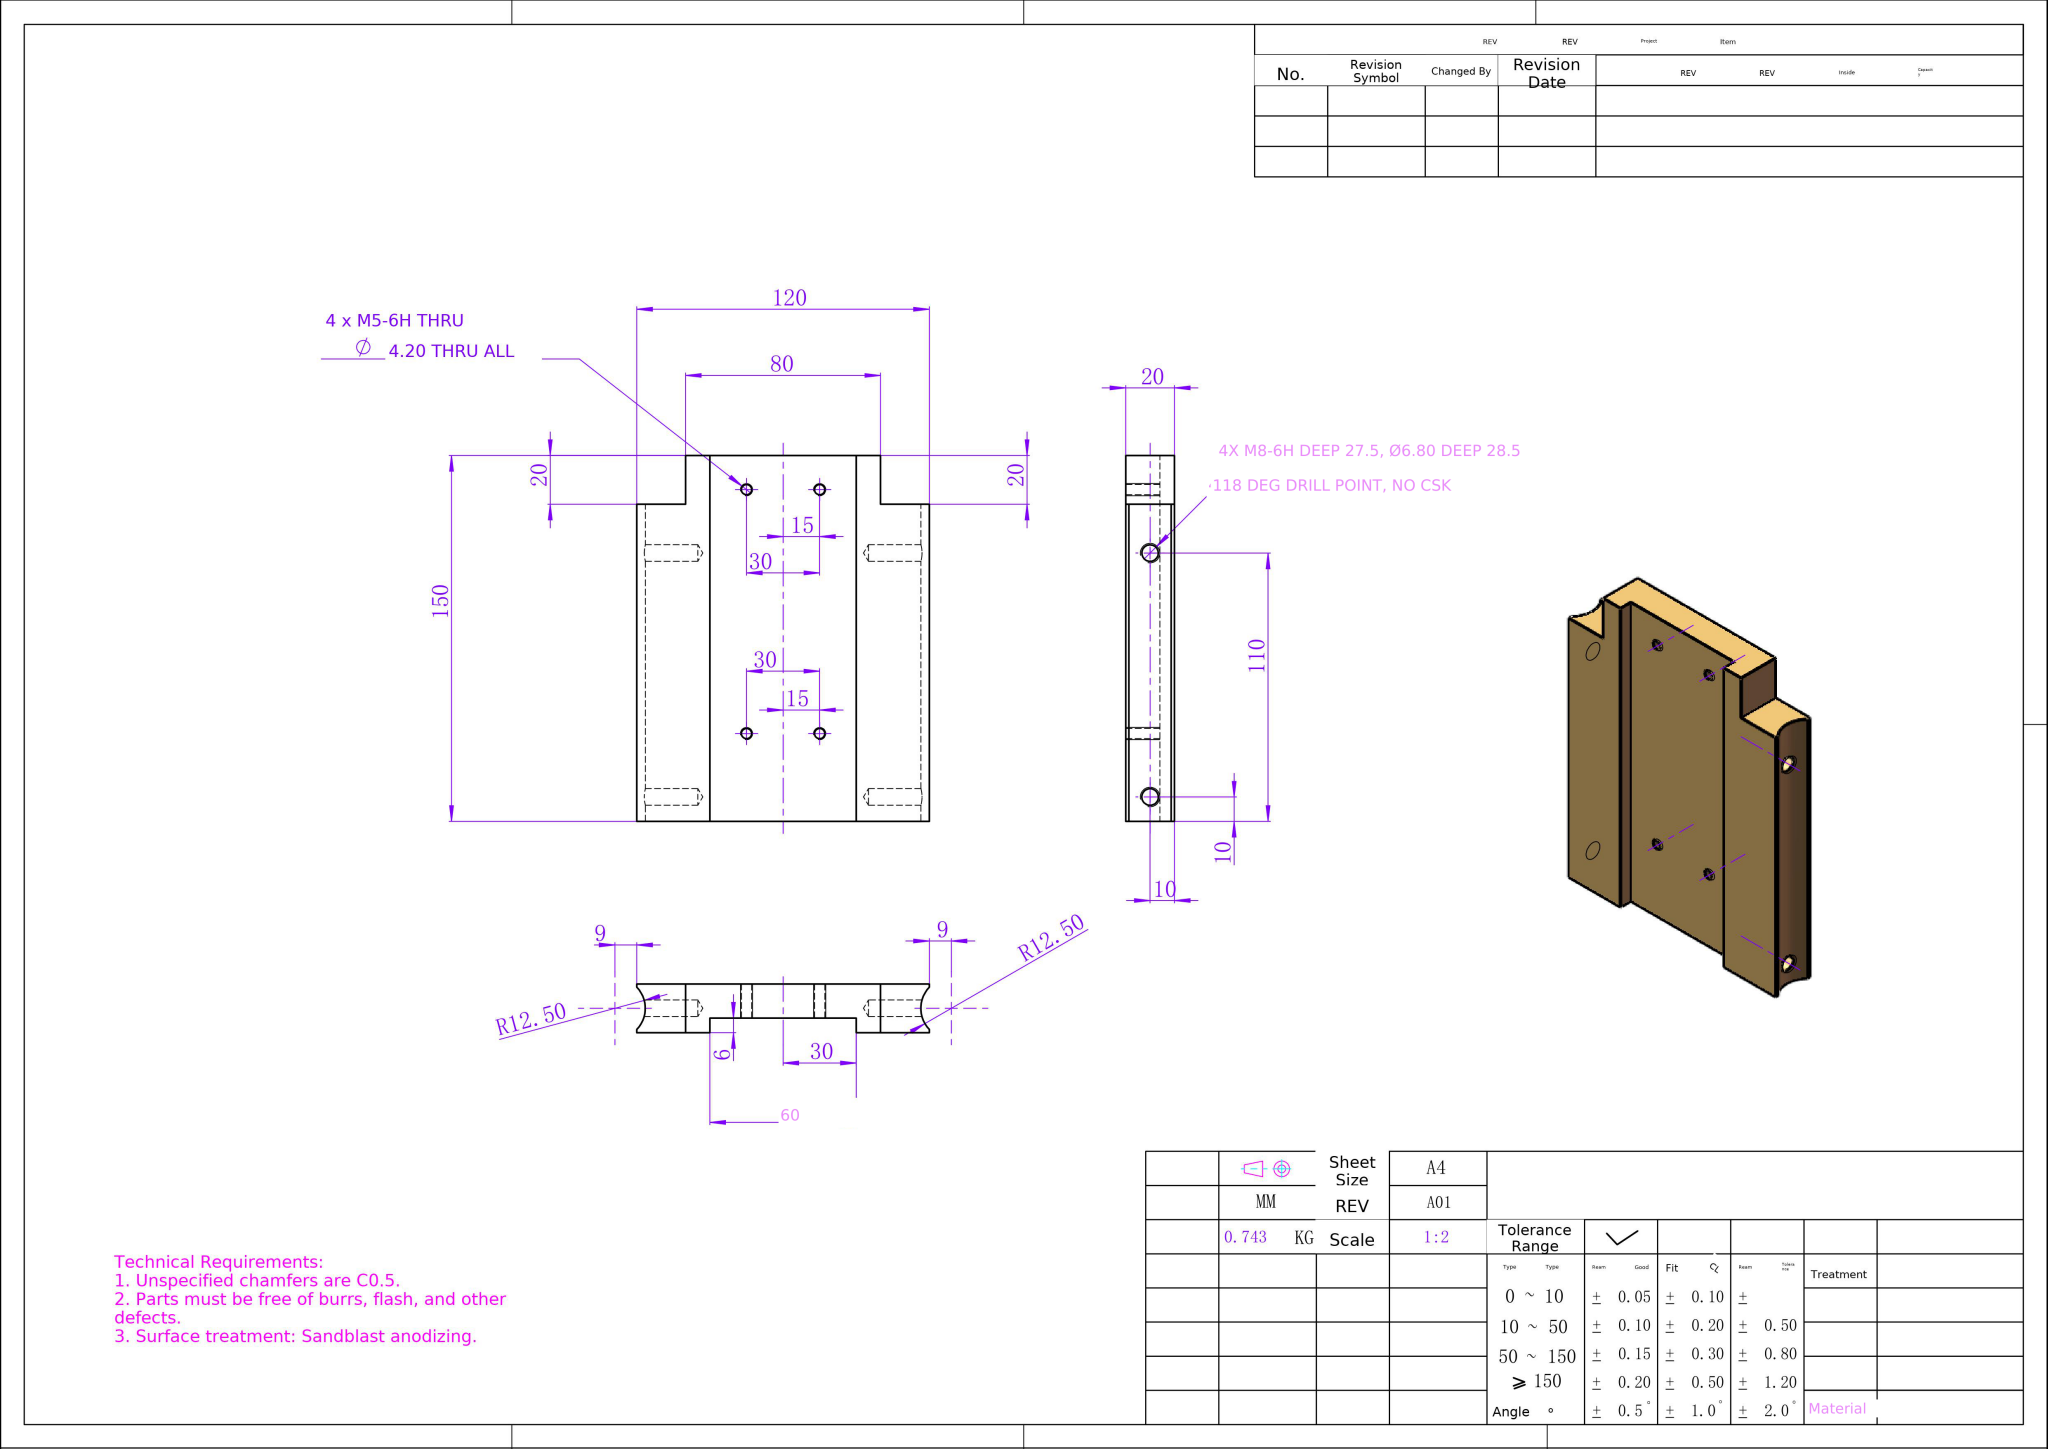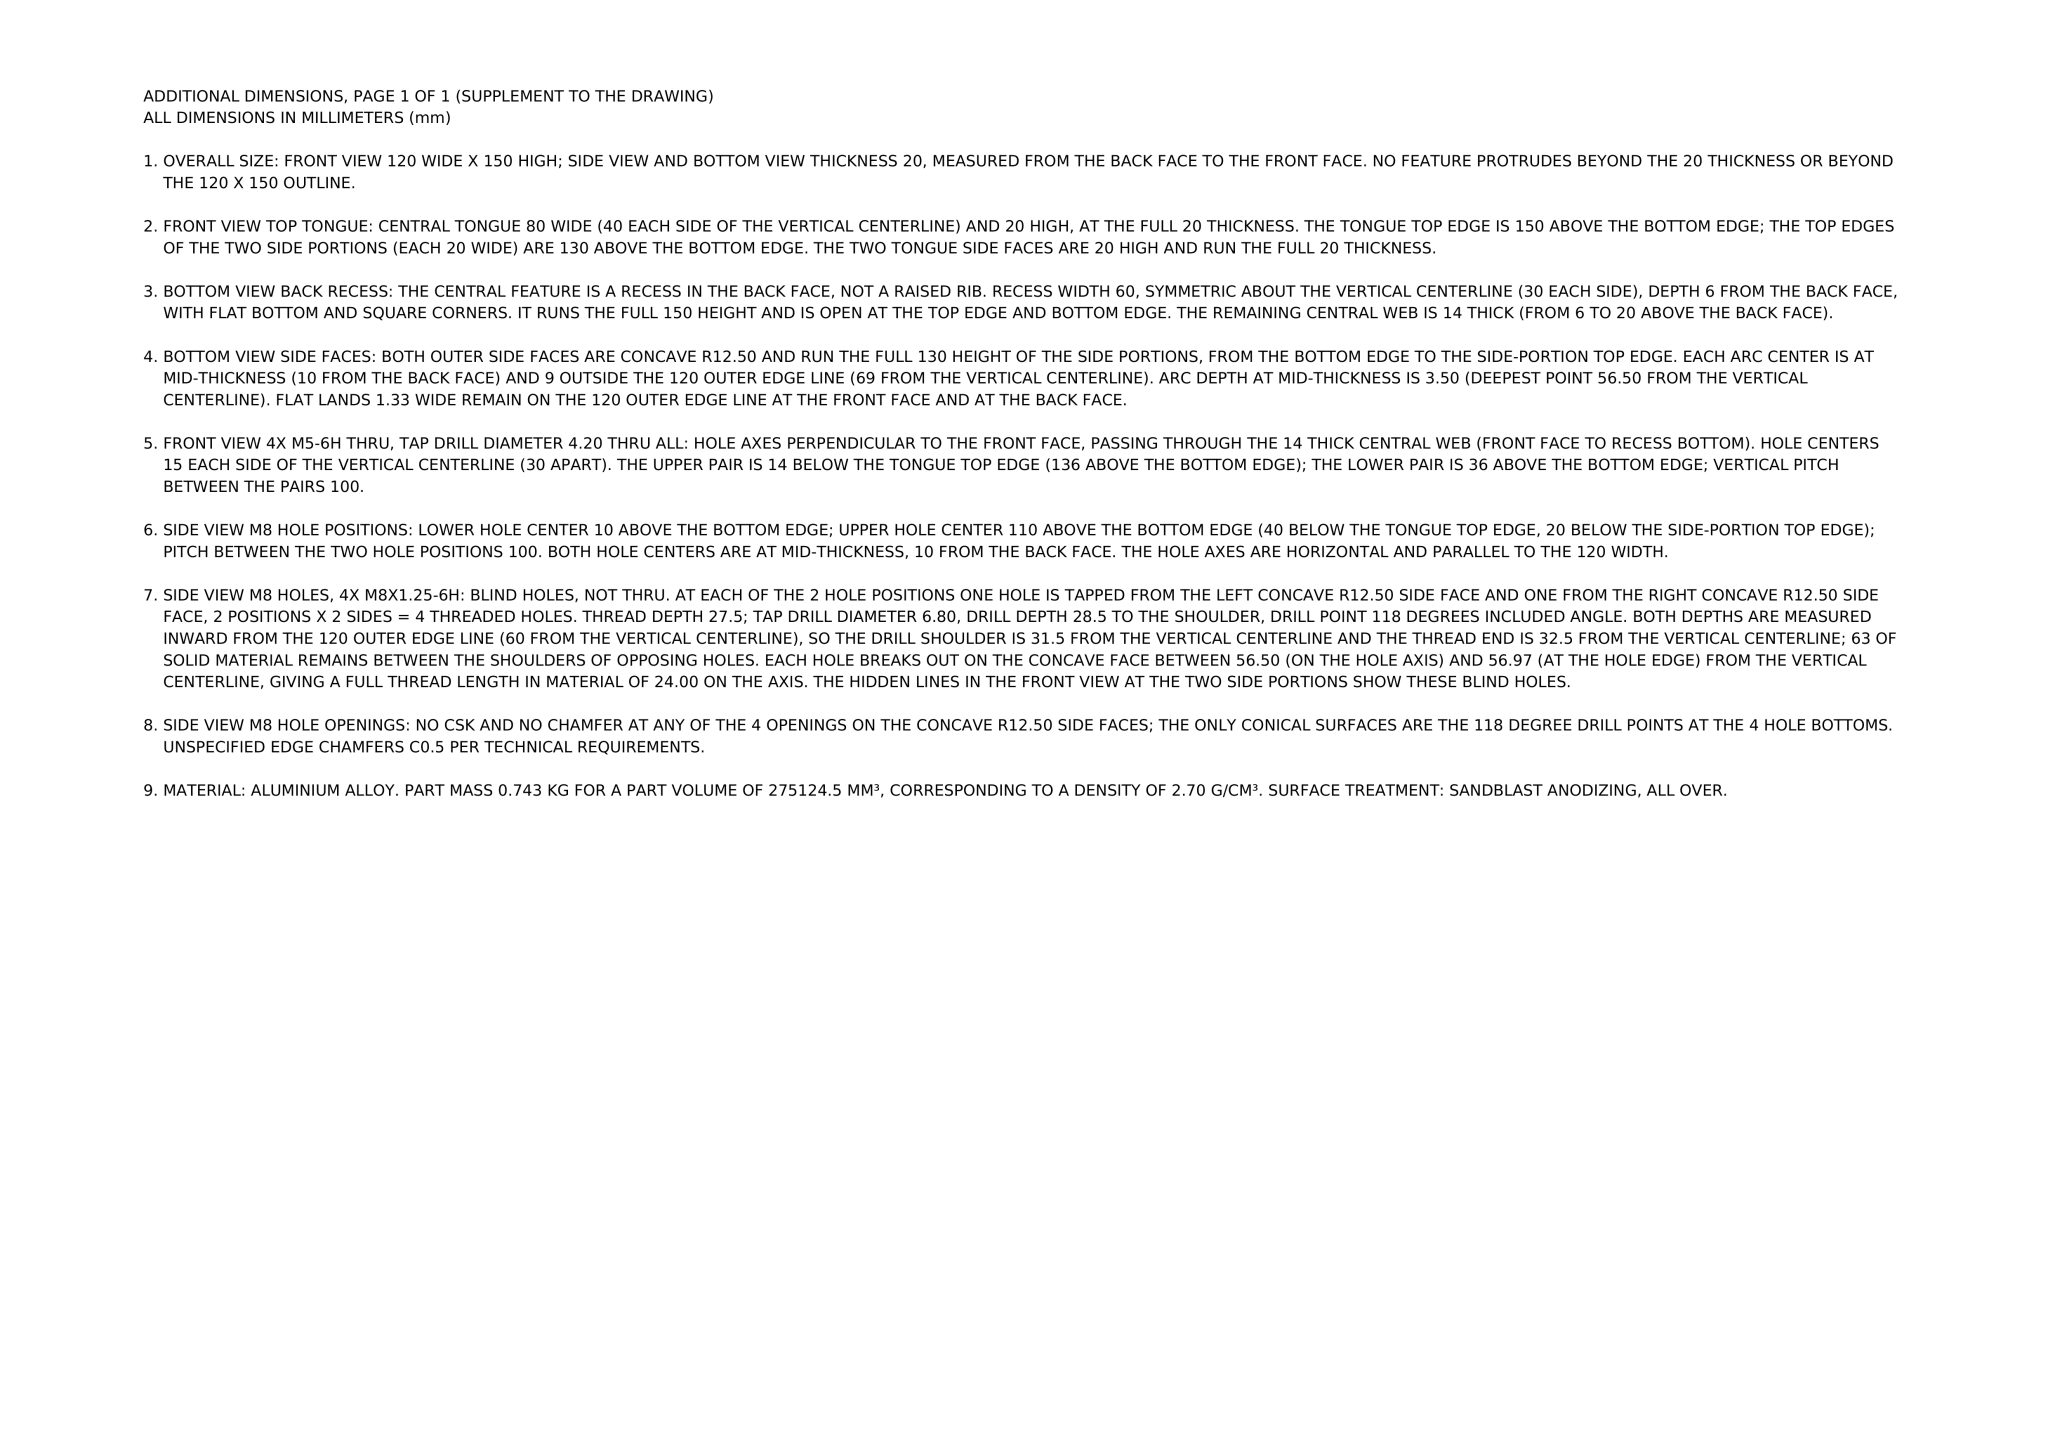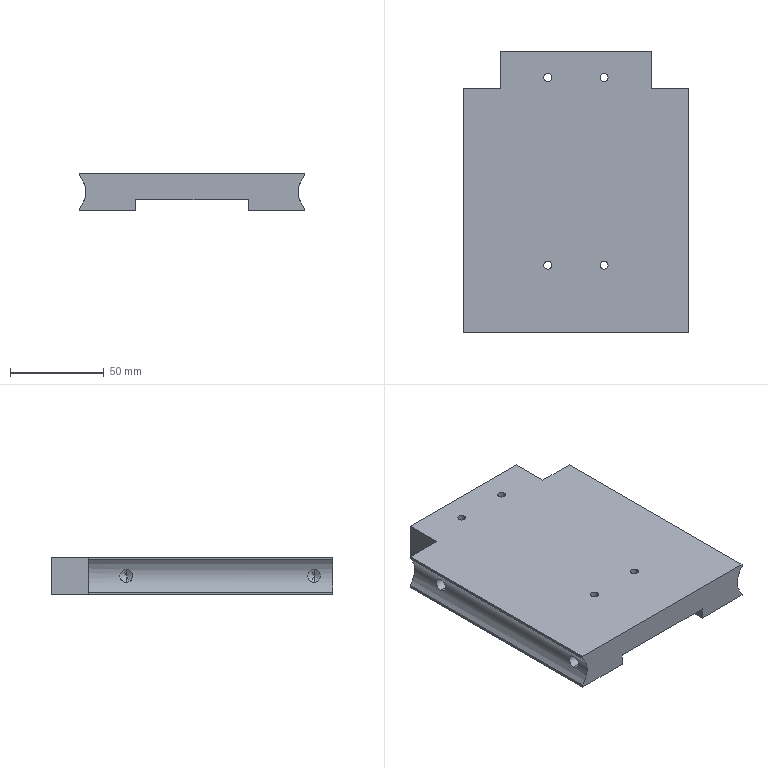Part | NX | mm | 1 solid | 42 faces | box 120 x 150 x 20 mm | volume 275124 mm3 | cylinder 18 | plane 16 | cone 8 | commonest cylinder face diameters 6.8 x8 4.2 x8 25 x2